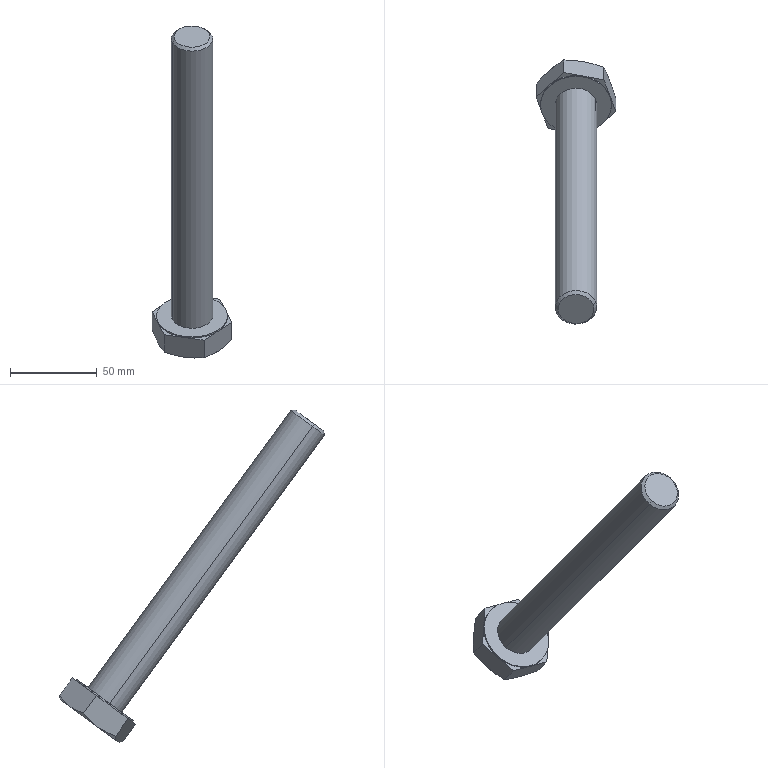Component | SolidWorks | hex structural bolt gradec short_iso-4 | 1 solid | 27 faces | box 46.18 x 152.88 x 191.78 mm | volume 112034 mm3 | plane 15 | cone 8 | cylinder 4 | commonest cylinder face diameters 41 x2 24 x2
STEP:
#1=CARTESIAN_POINT('',(-39.692,28.73,8.663));
#2=VERTEX_POINT('',#1);
#3=CARTESIAN_POINT('',(-38.151,29.116,8.946));
#4=VERTEX_POINT('',#3);
#5=CARTESIAN_POINT('',(-38.921,28.923,8.805));
#6=DIRECTION('',(0.,-0.5907,0.8069));
#7=DIRECTION('',(-0.9549,-0.2396,-0.1754));
#8=AXIS2_PLACEMENT_3D('',#5,#6,#7);
#9=CIRCLE('',#8,0.8071);
#10=EDGE_CURVE('',#2,#4,#9,.T.);
#11=ORIENTED_EDGE('',*,*,#10,.F.);
#12=CARTESIAN_POINT('',(-39.692,28.748,8.638));
#13=VERTEX_POINT('',#12);
#14=CARTESIAN_POINT('',(-39.692,29.079,8.187));
#15=DIRECTION('',(-0.,0.5907,-0.8069));
#16=VECTOR('',#15,39.37);
#17=LINE('',#14,#16);
#18=EDGE_CURVE('',#2,#13,#17,.T.);
#19=ORIENTED_EDGE('',*,*,#18,.T.);
#20=CARTESIAN_POINT('',(-39.099,28.307,8.314));
#21=VERTEX_POINT('',#20);
#22=CARTESIAN_POINT('',(-38.921,28.942,8.779));
#23=DIRECTION('',(-0.,0.5907,-0.8069));
#24=DIRECTION('',(0.9549,0.2396,0.1754));
#25=AXIS2_PLACEMENT_3D('',#22,#23,#24);
#26=CIRCLE('',#25,0.8071);
#27=EDGE_CURVE('',#21,#13,#26,.T.);
#28=ORIENTED_EDGE('',*,*,#27,.F.);
#29=CARTESIAN_POINT('',(-38.328,28.5,8.456));
#30=VERTEX_POINT('',#29);
#31=CARTESIAN_POINT('',(-38.921,28.942,8.779));
#32=DIRECTION('',(-0.,0.5907,-0.8069));
#33=DIRECTION('',(0.9549,0.2396,0.1754));
#34=AXIS2_PLACEMENT_3D('',#31,#32,#33);
#35=CIRCLE('',#34,0.8071);
#36=EDGE_CURVE('',#30,#21,#35,.T.);
#37=ORIENTED_EDGE('',*,*,#36,.F.);
#38=CARTESIAN_POINT('',(-38.151,29.135,8.921));
#39=VERTEX_POINT('',#38);
#40=CARTESIAN_POINT('',(-38.921,28.942,8.779));
#41=DIRECTION('',(-0.,0.5907,-0.8069));
#42=DIRECTION('',(0.9549,0.2396,0.1754));
#43=AXIS2_PLACEMENT_3D('',#40,#41,#42);
#44=CIRCLE('',#43,0.8071);
#45=EDGE_CURVE('',#39,#30,#44,.T.);
#46=ORIENTED_EDGE('',*,*,#45,.F.);
#47=CARTESIAN_POINT('',(-38.151,29.465,8.47));
#48=DIRECTION('',(-0.,0.5907,-0.8069));
#49=VECTOR('',#48,39.37);
#50=LINE('',#47,#49);
#51=EDGE_CURVE('',#4,#39,#50,.T.);
#52=ORIENTED_EDGE('',*,*,#51,.F.);
#53=EDGE_LOOP('',(#11,#19,#28,#37,#46,#52));
#54=FACE_OUTER_BOUND('',#53,.T.);
#55=CARTESIAN_POINT('',(-38.921,29.272,8.328));
#56=DIRECTION('',(-0.,0.5907,-0.8069));
#57=DIRECTION('',(0.9549,0.2396,0.1754));
#58=AXIS2_PLACEMENT_3D('',#55,#56,#57);
#59=CYLINDRICAL_SURFACE('',#58,0.8071);
#60=ADVANCED_FACE('',(#54),#59,.T.);
#61=CARTESIAN_POINT('',(-38.532,24.369,15.229));
#62=VERTEX_POINT('',#61);
#63=CARTESIAN_POINT('',(-39.31,24.174,15.086));
#64=VERTEX_POINT('',#63);
#65=CARTESIAN_POINT('',(-38.921,24.272,15.158));
#66=DIRECTION('',(-0.,0.5907,-0.8069));
#67=DIRECTION('',(0.9549,0.2396,0.1754));
#68=AXIS2_PLACEMENT_3D('',#65,#66,#67);
#69=CIRCLE('',#68,0.4076);
#70=EDGE_CURVE('',#62,#64,#69,.T.);
#71=ORIENTED_EDGE('',*,*,#70,.T.);
#72=CARTESIAN_POINT('',(-39.372,24.197,15.023));
#73=VERTEX_POINT('',#72);
#74=CARTESIAN_POINT('',(-39.31,24.174,15.086));
#75=DIRECTION('',(-0.6752,0.2483,-0.6946));
#76=VECTOR('',#75,39.37);
#77=LINE('',#74,#76);
#78=EDGE_CURVE('',#64,#73,#77,.T.);
#79=ORIENTED_EDGE('',*,*,#78,.T.);
#80=CARTESIAN_POINT('',(-38.47,24.423,15.188));
#81=VERTEX_POINT('',#80);
#82=CARTESIAN_POINT('',(-38.921,24.31,15.105));
#83=DIRECTION('',(-0.,0.5907,-0.8069));
#84=DIRECTION('',(0.9549,0.2396,0.1754));
#85=AXIS2_PLACEMENT_3D('',#82,#83,#84);
#86=CIRCLE('',#85,0.4724);
#87=EDGE_CURVE('',#81,#73,#86,.T.);
#88=ORIENTED_EDGE('',*,*,#87,.F.);
#89=CARTESIAN_POINT('',(-38.532,24.369,15.229));
#90=DIRECTION('',(0.6752,0.5871,-0.4465));
#91=VECTOR('',#90,39.37);
#92=LINE('',#89,#91);
#93=EDGE_CURVE('',#62,#81,#92,.T.);
#94=ORIENTED_EDGE('',*,*,#93,.F.);
#95=EDGE_LOOP('',(#71,#79,#88,#94));
#96=FACE_OUTER_BOUND('',#95,.T.);
#97=CARTESIAN_POINT('',(-38.921,24.272,15.158));
#98=DIRECTION('',(-0.,0.5907,-0.8069));
#99=DIRECTION('',(0.9549,0.2396,0.1754));
#100=AXIS2_PLACEMENT_3D('',#97,#98,#99);
#101=CONICAL_SURFACE('',#100,0.4076,0.7854);
#102=ADVANCED_FACE('',(#96),#101,.T.);
#103=ORIENTED_EDGE('',*,*,#87,.T.);
#104=CARTESIAN_POINT('',(-39.372,28.81,8.722));
#105=VERTEX_POINT('',#104);
#106=CARTESIAN_POINT('',(-39.372,29.159,8.245));
#107=DIRECTION('',(-0.,0.5907,-0.8069));
#108=VECTOR('',#107,39.37);
#109=LINE('',#106,#108);
#110=EDGE_CURVE('',#73,#105,#109,.T.);
#111=ORIENTED_EDGE('',*,*,#110,.T.);
#112=CARTESIAN_POINT('',(-38.47,29.036,8.887));
#113=VERTEX_POINT('',#112);
#114=CARTESIAN_POINT('',(-38.921,28.923,8.805));
#115=DIRECTION('',(-0.,0.5907,-0.8069));
#116=DIRECTION('',(-0.9549,-0.2396,-0.1754));
#117=AXIS2_PLACEMENT_3D('',#114,#115,#116);
#118=CIRCLE('',#117,0.4724);
#119=EDGE_CURVE('',#113,#105,#118,.T.);
#120=ORIENTED_EDGE('',*,*,#119,.F.);
#121=CARTESIAN_POINT('',(-38.47,29.385,8.411));
#122=DIRECTION('',(-0.,0.5907,-0.8069));
#123=VECTOR('',#122,39.37);
#124=LINE('',#121,#123);
#125=EDGE_CURVE('',#81,#113,#124,.T.);
#126=ORIENTED_EDGE('',*,*,#125,.F.);
#127=EDGE_LOOP('',(#103,#111,#120,#126));
#128=FACE_OUTER_BOUND('',#127,.T.);
#129=CARTESIAN_POINT('',(-38.921,29.272,8.328));
#130=DIRECTION('',(-0.,0.5907,-0.8069));
#131=DIRECTION('',(0.9549,0.2396,0.1754));
#132=AXIS2_PLACEMENT_3D('',#129,#130,#131);
#133=CYLINDRICAL_SURFACE('',#132,0.4724);
#134=ADVANCED_FACE('',(#128),#133,.T.);
#135=ORIENTED_EDGE('',*,*,#119,.T.);
#136=CARTESIAN_POINT('',(-38.921,28.923,8.805));
#137=DIRECTION('',(-0.,0.5907,-0.8069));
#138=DIRECTION('',(-0.9549,-0.2396,-0.1754));
#139=AXIS2_PLACEMENT_3D('',#136,#137,#138);
#140=CIRCLE('',#139,0.4724);
#141=EDGE_CURVE('',#105,#113,#140,.T.);
#142=ORIENTED_EDGE('',*,*,#141,.T.);
#143=EDGE_LOOP('',(#135,#142));
#144=FACE_BOUND('',#143,.T.);
#145=CARTESIAN_POINT('',(-38.921,28.923,8.805));
#146=DIRECTION('',(0.,-0.5907,0.8069));
#147=DIRECTION('',(-0.9549,-0.2396,-0.1754));
#148=AXIS2_PLACEMENT_3D('',#145,#146,#147);
#149=CIRCLE('',#148,0.8071);
#150=EDGE_CURVE('',#4,#2,#149,.T.);
#151=ORIENTED_EDGE('',*,*,#150,.T.);
#152=ORIENTED_EDGE('',*,*,#10,.T.);
#153=EDGE_LOOP('',(#151,#152));
#154=FACE_OUTER_BOUND('',#153,.T.);
#155=CARTESIAN_POINT('',(-38.645,28.205,8.279));
#156=DIRECTION('',(0.,-0.5907,0.8069));
#157=DIRECTION('',(-0.9549,-0.2396,-0.1754));
#158=AXIS2_PLACEMENT_3D('',#155,#156,#157);
#159=PLANE('',#158);
#160=ADVANCED_FACE('',(#144,#154),#159,.T.);
#161=ORIENTED_EDGE('',*,*,#110,.F.);
#162=CARTESIAN_POINT('',(-38.921,24.31,15.105));
#163=DIRECTION('',(-0.,0.5907,-0.8069));
#164=DIRECTION('',(0.9549,0.2396,0.1754));
#165=AXIS2_PLACEMENT_3D('',#162,#163,#164);
#166=CIRCLE('',#165,0.4724);
#167=EDGE_CURVE('',#73,#81,#166,.T.);
#168=ORIENTED_EDGE('',*,*,#167,.T.);
#169=ORIENTED_EDGE('',*,*,#125,.T.);
#170=ORIENTED_EDGE('',*,*,#141,.F.);
#171=EDGE_LOOP('',(#161,#168,#169,#170));
#172=FACE_OUTER_BOUND('',#171,.T.);
#173=CARTESIAN_POINT('',(-38.921,29.272,8.328));
#174=DIRECTION('',(-0.,0.5907,-0.8069));
#175=DIRECTION('',(0.9549,0.2396,0.1754));
#176=AXIS2_PLACEMENT_3D('',#173,#174,#175);
#177=CYLINDRICAL_SURFACE('',#176,0.4724);
#178=ADVANCED_FACE('',(#172),#177,.T.);
#179=ORIENTED_EDGE('',*,*,#78,.F.);
#180=CARTESIAN_POINT('',(-38.921,24.272,15.158));
#181=DIRECTION('',(-0.,0.5907,-0.8069));
#182=DIRECTION('',(0.9549,0.2396,0.1754));
#183=AXIS2_PLACEMENT_3D('',#180,#181,#182);
#184=CIRCLE('',#183,0.4076);
#185=EDGE_CURVE('',#64,#62,#184,.T.);
#186=ORIENTED_EDGE('',*,*,#185,.T.);
#187=ORIENTED_EDGE('',*,*,#93,.T.);
#188=ORIENTED_EDGE('',*,*,#167,.F.);
#189=EDGE_LOOP('',(#179,#186,#187,#188));
#190=FACE_OUTER_BOUND('',#189,.T.);
#191=CARTESIAN_POINT('',(-38.921,24.272,15.158));
#192=DIRECTION('',(-0.,0.5907,-0.8069));
#193=DIRECTION('',(0.9549,0.2396,0.1754));
#194=AXIS2_PLACEMENT_3D('',#191,#192,#193);
#195=CONICAL_SURFACE('',#194,0.4076,0.7854);
#196=ADVANCED_FACE('',(#190),#195,.T.);
#197=ORIENTED_EDGE('',*,*,#70,.F.);
#198=ORIENTED_EDGE('',*,*,#185,.F.);
#199=EDGE_LOOP('',(#197,#198));
#200=FACE_OUTER_BOUND('',#199,.T.);
#201=CARTESIAN_POINT('',(-38.921,24.272,15.158));
#202=DIRECTION('',(-0.,0.5907,-0.8069));
#203=DIRECTION('',(0.9549,0.2396,0.1754));
#204=AXIS2_PLACEMENT_3D('',#201,#202,#203);
#205=PLANE('',#204);
#206=ADVANCED_FACE('',(#200),#205,.F.);
#207=CARTESIAN_POINT('',(-39.554,28.389,8.375));
#208=VERTEX_POINT('',#207);
#209=CARTESIAN_POINT('',(-39.554,28.389,8.375));
#210=DIRECTION('',(0.9754,-0.1778,-0.1301));
#211=VECTOR('',#210,39.37);
#212=LINE('',#209,#211);
#213=EDGE_CURVE('',#208,#21,#212,.T.);
#214=ORIENTED_EDGE('',*,*,#213,.T.);
#215=ORIENTED_EDGE('',*,*,#27,.T.);
#216=CARTESIAN_POINT('',(-39.554,28.389,8.375));
#217=DIRECTION('',(0.2969,-0.7705,-0.5641));
#218=VECTOR('',#217,39.37);
#219=LINE('',#216,#218);
#220=EDGE_CURVE('',#13,#208,#219,.T.);
#221=ORIENTED_EDGE('',*,*,#220,.T.);
#222=EDGE_LOOP('',(#214,#215,#221));
#223=FACE_OUTER_BOUND('',#222,.T.);
#224=CARTESIAN_POINT('',(-38.682,28.32,8.324));
#225=DIRECTION('',(0.,-0.5907,0.8069));
#226=DIRECTION('',(-0.9549,-0.2396,-0.1754));
#227=AXIS2_PLACEMENT_3D('',#224,#225,#226);
#228=PLANE('',#227);
#229=ADVANCED_FACE('',(#223),#228,.T.);
#230=CARTESIAN_POINT('',(-38.645,28.224,8.253));
#231=VERTEX_POINT('',#230);
#232=CARTESIAN_POINT('',(-39.554,28.389,8.375));
#233=DIRECTION('',(0.9754,-0.1778,-0.1301));
#234=VECTOR('',#233,39.37);
#235=LINE('',#232,#234);
#236=EDGE_CURVE('',#21,#231,#235,.T.);
#237=ORIENTED_EDGE('',*,*,#236,.T.);
#238=CARTESIAN_POINT('',(-38.645,28.224,8.253));
#239=DIRECTION('',(0.6785,0.5927,0.434));
#240=VECTOR('',#239,39.37);
#241=LINE('',#238,#240);
#242=EDGE_CURVE('',#231,#30,#241,.T.);
#243=ORIENTED_EDGE('',*,*,#242,.T.);
#244=ORIENTED_EDGE('',*,*,#36,.T.);
#245=EDGE_LOOP('',(#237,#243,#244));
#246=FACE_OUTER_BOUND('',#245,.T.);
#247=CARTESIAN_POINT('',(-38.682,28.32,8.324));
#248=DIRECTION('',(0.,-0.5907,0.8069));
#249=DIRECTION('',(-0.9549,-0.2396,-0.1754));
#250=AXIS2_PLACEMENT_3D('',#247,#248,#249);
#251=PLANE('',#250);
#252=ADVANCED_FACE('',(#246),#251,.T.);
#253=CARTESIAN_POINT('',(-38.012,28.776,8.658));
#254=VERTEX_POINT('',#253);
#255=CARTESIAN_POINT('',(-38.645,28.224,8.253));
#256=DIRECTION('',(0.6785,0.5927,0.434));
#257=VECTOR('',#256,39.37);
#258=LINE('',#255,#257);
#259=EDGE_CURVE('',#30,#254,#258,.T.);
#260=ORIENTED_EDGE('',*,*,#259,.T.);
#261=CARTESIAN_POINT('',(-38.012,28.776,8.658));
#262=DIRECTION('',(-0.2969,0.7705,0.5641));
#263=VECTOR('',#262,39.37);
#264=LINE('',#261,#263);
#265=EDGE_CURVE('',#254,#39,#264,.T.);
#266=ORIENTED_EDGE('',*,*,#265,.T.);
#267=ORIENTED_EDGE('',*,*,#45,.T.);
#268=EDGE_LOOP('',(#260,#266,#267));
#269=FACE_OUTER_BOUND('',#268,.T.);
#270=CARTESIAN_POINT('',(-38.682,28.32,8.324));
#271=DIRECTION('',(0.,-0.5907,0.8069));
#272=DIRECTION('',(-0.9549,-0.2396,-0.1754));
#273=AXIS2_PLACEMENT_3D('',#270,#271,#272);
#274=PLANE('',#273);
#275=ADVANCED_FACE('',(#269),#274,.T.);
#276=CARTESIAN_POINT('',(-38.289,29.494,9.184));
#277=VERTEX_POINT('',#276);
#278=CARTESIAN_POINT('',(-38.012,28.776,8.658));
#279=DIRECTION('',(-0.2969,0.7705,0.5641));
#280=VECTOR('',#279,39.37);
#281=LINE('',#278,#280);
#282=EDGE_CURVE('',#39,#277,#281,.T.);
#283=ORIENTED_EDGE('',*,*,#282,.T.);
#284=CARTESIAN_POINT('',(-38.743,29.577,9.244));
#285=VERTEX_POINT('',#284);
#286=CARTESIAN_POINT('',(-39.198,29.66,9.305));
#287=DIRECTION('',(-0.9754,0.1778,0.1301));
#288=VECTOR('',#287,39.37);
#289=LINE('',#286,#288);
#290=EDGE_CURVE('',#277,#285,#289,.T.);
#291=ORIENTED_EDGE('',*,*,#290,.T.);
#292=CARTESIAN_POINT('',(-38.921,28.942,8.779));
#293=DIRECTION('',(-0.,0.5907,-0.8069));
#294=DIRECTION('',(0.9549,0.2396,0.1754));
#295=AXIS2_PLACEMENT_3D('',#292,#293,#294);
#296=CIRCLE('',#295,0.8071);
#297=EDGE_CURVE('',#285,#39,#296,.T.);
#298=ORIENTED_EDGE('',*,*,#297,.T.);
#299=EDGE_LOOP('',(#283,#291,#298));
#300=FACE_OUTER_BOUND('',#299,.T.);
#301=CARTESIAN_POINT('',(-38.682,28.32,8.324));
#302=DIRECTION('',(0.,-0.5907,0.8069));
#303=DIRECTION('',(-0.9549,-0.2396,-0.1754));
#304=AXIS2_PLACEMENT_3D('',#301,#302,#303);
#305=PLANE('',#304);
#306=ADVANCED_FACE('',(#300),#305,.T.);
#307=CARTESIAN_POINT('',(-39.198,29.66,9.305));
#308=VERTEX_POINT('',#307);
#309=CARTESIAN_POINT('',(-39.198,29.66,9.305));
#310=DIRECTION('',(-0.9754,0.1778,0.1301));
#311=VECTOR('',#310,39.37);
#312=LINE('',#309,#311);
#313=EDGE_CURVE('',#285,#308,#312,.T.);
#314=ORIENTED_EDGE('',*,*,#313,.T.);
#315=CARTESIAN_POINT('',(-39.514,29.384,9.103));
#316=VERTEX_POINT('',#315);
#317=CARTESIAN_POINT('',(-39.83,29.107,8.901));
#318=DIRECTION('',(-0.6785,-0.5927,-0.434));
#319=VECTOR('',#318,39.37);
#320=LINE('',#317,#319);
#321=EDGE_CURVE('',#308,#316,#320,.T.);
#322=ORIENTED_EDGE('',*,*,#321,.T.);
#323=CARTESIAN_POINT('',(-38.921,28.942,8.779));
#324=DIRECTION('',(-0.,0.5907,-0.8069));
#325=DIRECTION('',(0.9549,0.2396,0.1754));
#326=AXIS2_PLACEMENT_3D('',#323,#324,#325);
#327=CIRCLE('',#326,0.8071);
#328=EDGE_CURVE('',#316,#285,#327,.T.);
#329=ORIENTED_EDGE('',*,*,#328,.T.);
#330=EDGE_LOOP('',(#314,#322,#329));
#331=FACE_OUTER_BOUND('',#330,.T.);
#332=CARTESIAN_POINT('',(-38.682,28.32,8.324));
#333=DIRECTION('',(0.,-0.5907,0.8069));
#334=DIRECTION('',(-0.9549,-0.2396,-0.1754));
#335=AXIS2_PLACEMENT_3D('',#332,#333,#334);
#336=PLANE('',#335);
#337=ADVANCED_FACE('',(#331),#336,.T.);
#338=CARTESIAN_POINT('',(-39.83,29.107,8.901));
#339=VERTEX_POINT('',#338);
#340=CARTESIAN_POINT('',(-39.83,29.107,8.901));
#341=DIRECTION('',(-0.6785,-0.5927,-0.434));
#342=VECTOR('',#341,39.37);
#343=LINE('',#340,#342);
#344=EDGE_CURVE('',#316,#339,#343,.T.);
#345=ORIENTED_EDGE('',*,*,#344,.T.);
#346=CARTESIAN_POINT('',(-39.554,28.389,8.375));
#347=DIRECTION('',(0.2969,-0.7705,-0.5641));
#348=VECTOR('',#347,39.37);
#349=LINE('',#346,#348);
#350=EDGE_CURVE('',#339,#13,#349,.T.);
#351=ORIENTED_EDGE('',*,*,#350,.T.);
#352=CARTESIAN_POINT('',(-38.921,28.942,8.779));
#353=DIRECTION('',(-0.,0.5907,-0.8069));
#354=DIRECTION('',(0.9549,0.2396,0.1754));
#355=AXIS2_PLACEMENT_3D('',#352,#353,#354);
#356=CIRCLE('',#355,0.8071);
#357=EDGE_CURVE('',#13,#316,#356,.T.);
#358=ORIENTED_EDGE('',*,*,#357,.T.);
#359=EDGE_LOOP('',(#345,#351,#358));
#360=FACE_OUTER_BOUND('',#359,.T.);
#361=CARTESIAN_POINT('',(-38.682,28.32,8.324));
#362=DIRECTION('',(0.,-0.5907,0.8069));
#363=DIRECTION('',(-0.9549,-0.2396,-0.1754));
#364=AXIS2_PLACEMENT_3D('',#361,#362,#363);
#365=PLANE('',#364);
#366=ADVANCED_FACE('',(#360),#365,.T.);
#367=ORIENTED_EDGE('',*,*,#18,.F.);
#368=ORIENTED_EDGE('',*,*,#150,.F.);
#369=ORIENTED_EDGE('',*,*,#51,.T.);
#370=ORIENTED_EDGE('',*,*,#297,.F.);
#371=ORIENTED_EDGE('',*,*,#328,.F.);
#372=ORIENTED_EDGE('',*,*,#357,.F.);
#373=EDGE_LOOP('',(#367,#368,#369,#370,#371,#372));
#374=FACE_OUTER_BOUND('',#373,.T.);
#375=CARTESIAN_POINT('',(-38.921,29.272,8.328));
#376=DIRECTION('',(-0.,0.5907,-0.8069));
#377=DIRECTION('',(0.9549,0.2396,0.1754));
#378=AXIS2_PLACEMENT_3D('',#375,#376,#377);
#379=CYLINDRICAL_SURFACE('',#378,0.8071);
#380=ADVANCED_FACE('',(#374),#379,.T.);
#381=CARTESIAN_POINT('',(-39.692,29.079,8.187));
#382=VERTEX_POINT('',#381);
#383=CARTESIAN_POINT('',(-39.099,28.637,7.863));
#384=VERTEX_POINT('',#383);
#385=CARTESIAN_POINT('',(-38.921,29.272,8.328));
#386=DIRECTION('',(0.,-0.5907,0.8069));
#387=DIRECTION('',(-0.9549,-0.2396,-0.1754));
#388=AXIS2_PLACEMENT_3D('',#385,#386,#387);
#389=CIRCLE('',#388,0.8071);
#390=EDGE_CURVE('',#382,#384,#389,.T.);
#391=ORIENTED_EDGE('',*,*,#390,.F.);
#392=CARTESIAN_POINT('',(-39.514,29.714,8.652));
#393=VERTEX_POINT('',#392);
#394=CARTESIAN_POINT('',(-38.921,29.272,8.328));
#395=DIRECTION('',(0.,-0.5907,0.8069));
#396=DIRECTION('',(-0.9549,-0.2396,-0.1754));
#397=AXIS2_PLACEMENT_3D('',#394,#395,#396);
#398=CIRCLE('',#397,0.8071);
#399=EDGE_CURVE('',#393,#382,#398,.T.);
#400=ORIENTED_EDGE('',*,*,#399,.F.);
#401=CARTESIAN_POINT('',(-38.743,29.907,8.793));
#402=VERTEX_POINT('',#401);
#403=CARTESIAN_POINT('',(-38.921,29.272,8.328));
#404=DIRECTION('',(0.,-0.5907,0.8069));
#405=DIRECTION('',(-0.9549,-0.2396,-0.1754));
#406=AXIS2_PLACEMENT_3D('',#403,#404,#405);
#407=CIRCLE('',#406,0.8071);
#408=EDGE_CURVE('',#402,#393,#407,.T.);
#409=ORIENTED_EDGE('',*,*,#408,.F.);
#410=CARTESIAN_POINT('',(-38.151,29.465,8.47));
#411=VERTEX_POINT('',#410);
#412=CARTESIAN_POINT('',(-38.921,29.272,8.328));
#413=DIRECTION('',(0.,-0.5907,0.8069));
#414=DIRECTION('',(-0.9549,-0.2396,-0.1754));
#415=AXIS2_PLACEMENT_3D('',#412,#413,#414);
#416=CIRCLE('',#415,0.8071);
#417=EDGE_CURVE('',#411,#402,#416,.T.);
#418=ORIENTED_EDGE('',*,*,#417,.F.);
#419=CARTESIAN_POINT('',(-38.328,28.83,8.005));
#420=VERTEX_POINT('',#419);
#421=CARTESIAN_POINT('',(-38.921,29.272,8.328));
#422=DIRECTION('',(-0.,0.5907,-0.8069));
#423=DIRECTION('',(0.9549,0.2396,0.1754));
#424=AXIS2_PLACEMENT_3D('',#421,#422,#423);
#425=CIRCLE('',#424,0.8071);
#426=EDGE_CURVE('',#411,#420,#425,.T.);
#427=ORIENTED_EDGE('',*,*,#426,.T.);
#428=CARTESIAN_POINT('',(-38.921,29.272,8.328));
#429=DIRECTION('',(0.,-0.5907,0.8069));
#430=DIRECTION('',(-0.9549,-0.2396,-0.1754));
#431=AXIS2_PLACEMENT_3D('',#428,#429,#430);
#432=CIRCLE('',#431,0.8071);
#433=EDGE_CURVE('',#384,#420,#432,.T.);
#434=ORIENTED_EDGE('',*,*,#433,.F.);
#435=EDGE_LOOP('',(#391,#400,#409,#418,#427,#434));
#436=FACE_OUTER_BOUND('',#435,.T.);
#437=CARTESIAN_POINT('',(-38.645,28.554,7.802));
#438=DIRECTION('',(0.,-0.5907,0.8069));
#439=DIRECTION('',(-0.9549,-0.2396,-0.1754));
#440=AXIS2_PLACEMENT_3D('',#437,#438,#439);
#441=PLANE('',#440);
#442=ADVANCED_FACE('',(#436),#441,.F.);
#443=CARTESIAN_POINT('',(-38.645,28.511,7.861));
#444=VERTEX_POINT('',#443);
#445=CARTESIAN_POINT('',(-38.328,28.83,8.005));
#446=CARTESIAN_POINT('',(-38.342,28.818,7.996));
#447=CARTESIAN_POINT('',(-38.355,28.806,7.988));
#448=CARTESIAN_POINT('',(-38.382,28.782,7.972));
#449=CARTESIAN_POINT('',(-38.395,28.77,7.964));
#450=CARTESIAN_POINT('',(-38.435,28.732,7.943));
#451=CARTESIAN_POINT('',(-38.462,28.706,7.93));
#452=CARTESIAN_POINT('',(-38.541,28.626,7.895));
#453=CARTESIAN_POINT('',(-38.593,28.569,7.876));
#454=CARTESIAN_POINT('',(-38.645,28.511,7.861));
#455=B_SPLINE_CURVE_WITH_KNOTS('',3,(#445,#446,#447,#448,#449,#450,#451,#452,#453,#454),.UNSPECIFIED.,.F.,.F.,(4,2,2,2,4),(0.01198,0.01347,0.01496,0.01794,0.02391),.UNSPECIFIED.);
#456=EDGE_CURVE('',#420,#444,#455,.T.);
#457=ORIENTED_EDGE('',*,*,#456,.T.);
#458=CARTESIAN_POINT('',(-38.645,28.511,7.861));
#459=CARTESIAN_POINT('',(-38.719,28.538,7.853));
#460=CARTESIAN_POINT('',(-38.794,28.562,7.848));
#461=CARTESIAN_POINT('',(-38.945,28.605,7.848));
#462=CARTESIAN_POINT('',(-39.022,28.623,7.853));
#463=CARTESIAN_POINT('',(-39.099,28.637,7.863));
#464=B_SPLINE_CURVE_WITH_KNOTS('',3,(#458,#459,#460,#461,#462,#463),.UNSPECIFIED.,.F.,.F.,(4,2,4),(0.00000024,0.005988,0.01198),.UNSPECIFIED.);
#465=EDGE_CURVE('',#444,#384,#464,.T.);
#466=ORIENTED_EDGE('',*,*,#465,.T.);
#467=ORIENTED_EDGE('',*,*,#433,.T.);
#468=EDGE_LOOP('',(#457,#466,#467));
#469=FACE_OUTER_BOUND('',#468,.T.);
#470=CARTESIAN_POINT('',(-38.921,29.272,8.328));
#471=DIRECTION('',(0.,-0.5907,0.8069));
#472=DIRECTION('',(-0.9549,-0.2396,-0.1754));
#473=AXIS2_PLACEMENT_3D('',#470,#471,#472);
#474=CONICAL_SURFACE('',#473,0.8071,1.047);
#475=ADVANCED_FACE('',(#469),#474,.T.);
#476=CARTESIAN_POINT('',(-38.012,29.064,8.265));
#477=VERTEX_POINT('',#476);
#478=CARTESIAN_POINT('',(-38.151,29.465,8.47));
#479=CARTESIAN_POINT('',(-38.139,29.435,8.447));
#480=CARTESIAN_POINT('',(-38.127,29.403,8.426));
#481=CARTESIAN_POINT('',(-38.104,29.338,8.387));
#482=CARTESIAN_POINT('',(-38.092,29.305,8.369));
#483=CARTESIAN_POINT('',(-38.057,29.204,8.318));
#484=CARTESIAN_POINT('',(-38.035,29.135,8.29));
#485=CARTESIAN_POINT('',(-38.012,29.064,8.265));
#486=B_SPLINE_CURVE_WITH_KNOTS('',3,(#478,#479,#480,#481,#482,#483,#484,#485),.UNSPECIFIED.,.F.,.F.,(4,2,2,4),(0.03354,0.03654,0.03953,0.04553),.UNSPECIFIED.);
#487=EDGE_CURVE('',#411,#477,#486,.T.);
#488=ORIENTED_EDGE('',*,*,#487,.T.);
#489=CARTESIAN_POINT('',(-38.012,29.064,8.265));
#490=CARTESIAN_POINT('',(-38.064,29.032,8.214));
#491=CARTESIAN_POINT('',(-38.116,28.997,8.166));
#492=CARTESIAN_POINT('',(-38.221,28.92,8.079));
#493=CARTESIAN_POINT('',(-38.275,28.877,8.039));
#494=CARTESIAN_POINT('',(-38.328,28.83,8.005));
#495=B_SPLINE_CURVE_WITH_KNOTS('',3,(#489,#490,#491,#492,#493,#494),.UNSPECIFIED.,.F.,.F.,(4,2,4),(0.00000024,0.005988,0.01198),.UNSPECIFIED.);
#496=EDGE_CURVE('',#477,#420,#495,.T.);
#497=ORIENTED_EDGE('',*,*,#496,.T.);
#498=ORIENTED_EDGE('',*,*,#426,.F.);
#499=EDGE_LOOP('',(#488,#497,#498));
#500=FACE_OUTER_BOUND('',#499,.T.);
#501=CARTESIAN_POINT('',(-38.921,29.272,8.328));
#502=DIRECTION('',(0.,-0.5907,0.8069));
#503=DIRECTION('',(-0.9549,-0.2396,-0.1754));
#504=AXIS2_PLACEMENT_3D('',#501,#502,#503);
#505=CONICAL_SURFACE('',#504,0.8071,1.047);
#506=ADVANCED_FACE('',(#500),#505,.T.);
#507=CARTESIAN_POINT('',(-38.289,29.782,8.791));
#508=VERTEX_POINT('',#507);
#509=CARTESIAN_POINT('',(-38.289,29.782,8.791));
#510=CARTESIAN_POINT('',(-38.278,29.759,8.761));
#511=CARTESIAN_POINT('',(-38.266,29.735,8.731));
#512=CARTESIAN_POINT('',(-38.243,29.686,8.673));
#513=CARTESIAN_POINT('',(-38.232,29.661,8.645));
#514=CARTESIAN_POINT('',(-38.197,29.582,8.564));
#515=CARTESIAN_POINT('',(-38.174,29.526,8.514));
#516=CARTESIAN_POINT('',(-38.151,29.465,8.47));
#517=B_SPLINE_CURVE_WITH_KNOTS('',3,(#509,#510,#511,#512,#513,#514,#515,#516),.UNSPECIFIED.,.F.,.F.,(4,2,2,4),(0.02156,0.02456,0.02755,0.03354),.UNSPECIFIED.);
#518=EDGE_CURVE('',#508,#411,#517,.T.);
#519=ORIENTED_EDGE('',*,*,#518,.T.);
#520=ORIENTED_EDGE('',*,*,#417,.T.);
#521=CARTESIAN_POINT('',(-38.743,29.907,8.793));
#522=CARTESIAN_POINT('',(-38.724,29.904,8.791));
#523=CARTESIAN_POINT('',(-38.705,29.9,8.788));
#524=CARTESIAN_POINT('',(-38.666,29.892,8.785));
#525=CARTESIAN_POINT('',(-38.647,29.888,8.783));
#526=CARTESIAN_POINT('',(-38.589,29.874,8.779));
#527=CARTESIAN_POINT('',(-38.551,29.864,8.778));
#528=CARTESIAN_POINT('',(-38.438,29.833,8.778));
#529=CARTESIAN_POINT('',(-38.363,29.808,8.783));
#530=CARTESIAN_POINT('',(-38.289,29.782,8.791));
#531=B_SPLINE_CURVE_WITH_KNOTS('',3,(#521,#522,#523,#524,#525,#526,#527,#528,#529,#530),.UNSPECIFIED.,.F.,.F.,(4,2,2,2,4),(0.01198,0.01347,0.01496,0.01794,0.02391),.UNSPECIFIED.);
#532=EDGE_CURVE('',#402,#508,#531,.T.);
#533=ORIENTED_EDGE('',*,*,#532,.T.);
#534=EDGE_LOOP('',(#519,#520,#533));
#535=FACE_OUTER_BOUND('',#534,.T.);
#536=CARTESIAN_POINT('',(-38.921,29.272,8.328));
#537=DIRECTION('',(0.,-0.5907,0.8069));
#538=DIRECTION('',(-0.9549,-0.2396,-0.1754));
#539=AXIS2_PLACEMENT_3D('',#536,#537,#538);
#540=CONICAL_SURFACE('',#539,0.8071,1.047);
#541=ADVANCED_FACE('',(#535),#540,.T.);
#542=CARTESIAN_POINT('',(-39.198,29.947,8.912));
#543=VERTEX_POINT('',#542);
#544=CARTESIAN_POINT('',(-39.198,29.947,8.912));
#545=CARTESIAN_POINT('',(-39.124,29.947,8.884));
#546=CARTESIAN_POINT('',(-39.049,29.944,8.86));
#547=CARTESIAN_POINT('',(-38.897,29.931,8.819));
#548=CARTESIAN_POINT('',(-38.821,29.921,8.804));
#549=CARTESIAN_POINT('',(-38.743,29.907,8.793));
#550=B_SPLINE_CURVE_WITH_KNOTS('',3,(#544,#545,#546,#547,#548,#549),.UNSPECIFIED.,.F.,.F.,(4,2,4),(0.00000024,0.005988,0.01198),.UNSPECIFIED.);
#551=EDGE_CURVE('',#543,#402,#550,.T.);
#552=ORIENTED_EDGE('',*,*,#551,.T.);
#553=ORIENTED_EDGE('',*,*,#408,.T.);
#554=CARTESIAN_POINT('',(-39.514,29.714,8.652));
#555=CARTESIAN_POINT('',(-39.501,29.726,8.66));
#556=CARTESIAN_POINT('',(-39.487,29.737,8.669));
#557=CARTESIAN_POINT('',(-39.46,29.76,8.688));
#558=CARTESIAN_POINT('',(-39.447,29.77,8.697));
#559=CARTESIAN_POINT('',(-39.407,29.802,8.727));
#560=CARTESIAN_POINT('',(-39.381,29.823,8.748));
#561=CARTESIAN_POINT('',(-39.302,29.881,8.813));
#562=CARTESIAN_POINT('',(-39.25,29.915,8.861));
#563=CARTESIAN_POINT('',(-39.198,29.947,8.912));
#564=B_SPLINE_CURVE_WITH_KNOTS('',3,(#554,#555,#556,#557,#558,#559,#560,#561,#562,#563),.UNSPECIFIED.,.F.,.F.,(4,2,2,2,4),(0.01198,0.01347,0.01496,0.01794,0.02391),.UNSPECIFIED.);
#565=EDGE_CURVE('',#393,#543,#564,.T.);
#566=ORIENTED_EDGE('',*,*,#565,.T.);
#567=EDGE_LOOP('',(#552,#553,#566));
#568=FACE_OUTER_BOUND('',#567,.T.);
#569=CARTESIAN_POINT('',(-38.921,29.272,8.328));
#570=DIRECTION('',(0.,-0.5907,0.8069));
#571=DIRECTION('',(-0.9549,-0.2396,-0.1754));
#572=AXIS2_PLACEMENT_3D('',#569,#570,#571);
#573=CONICAL_SURFACE('',#572,0.8071,1.047);
#574=ADVANCED_FACE('',(#568),#573,.T.);
#575=CARTESIAN_POINT('',(-39.554,28.677,7.982));
#576=VERTEX_POINT('',#575);
#577=CARTESIAN_POINT('',(-39.099,28.637,7.863));
#578=CARTESIAN_POINT('',(-39.118,28.64,7.866));
#579=CARTESIAN_POINT('',(-39.138,28.644,7.869));
#580=CARTESIAN_POINT('',(-39.176,28.65,7.875));
#581=CARTESIAN_POINT('',(-39.196,28.652,7.879));
#582=CARTESIAN_POINT('',(-39.253,28.66,7.89));
#583=CARTESIAN_POINT('',(-39.291,28.664,7.899));
#584=CARTESIAN_POINT('',(-39.405,28.674,7.93));
#585=CARTESIAN_POINT('',(-39.479,28.676,7.954));
#586=CARTESIAN_POINT('',(-39.554,28.677,7.982));
#587=B_SPLINE_CURVE_WITH_KNOTS('',3,(#577,#578,#579,#580,#581,#582,#583,#584,#585,#586),.UNSPECIFIED.,.F.,.F.,(4,2,2,2,4),(0.01198,0.01347,0.01496,0.01794,0.02391),.UNSPECIFIED.);
#588=EDGE_CURVE('',#384,#576,#587,.T.);
#589=ORIENTED_EDGE('',*,*,#588,.T.);
#590=CARTESIAN_POINT('',(-39.554,28.677,7.982));
#591=CARTESIAN_POINT('',(-39.576,28.748,8.007));
#592=CARTESIAN_POINT('',(-39.599,28.817,8.035));
#593=CARTESIAN_POINT('',(-39.633,28.919,8.086));
#594=CARTESIAN_POINT('',(-39.645,28.952,8.104));
#595=CARTESIAN_POINT('',(-39.668,29.017,8.143));
#596=CARTESIAN_POINT('',(-39.68,29.048,8.164));
#597=CARTESIAN_POINT('',(-39.692,29.079,8.187));
#598=B_SPLINE_CURVE_WITH_KNOTS('',3,(#590,#591,#592,#593,#594,#595,#596,#597),.UNSPECIFIED.,.F.,.F.,(4,2,2,4),(0.0533,0.05929,0.06229,0.06529),.UNSPECIFIED.);
#599=EDGE_CURVE('',#576,#382,#598,.T.);
#600=ORIENTED_EDGE('',*,*,#599,.T.);
#601=ORIENTED_EDGE('',*,*,#390,.T.);
#602=EDGE_LOOP('',(#589,#600,#601));
#603=FACE_OUTER_BOUND('',#602,.T.);
#604=CARTESIAN_POINT('',(-38.921,29.272,8.328));
#605=DIRECTION('',(0.,-0.5907,0.8069));
#606=DIRECTION('',(-0.9549,-0.2396,-0.1754));
#607=AXIS2_PLACEMENT_3D('',#604,#605,#606);
#608=CONICAL_SURFACE('',#607,0.8071,1.047);
#609=ADVANCED_FACE('',(#603),#608,.T.);
#610=CARTESIAN_POINT('',(-39.83,29.395,8.508));
#611=VERTEX_POINT('',#610);
#612=CARTESIAN_POINT('',(-39.83,29.395,8.508));
#613=CARTESIAN_POINT('',(-39.779,29.453,8.523));
#614=CARTESIAN_POINT('',(-39.726,29.509,8.542));
#615=CARTESIAN_POINT('',(-39.621,29.616,8.589));
#616=CARTESIAN_POINT('',(-39.568,29.667,8.617));
#617=CARTESIAN_POINT('',(-39.514,29.714,8.652));
#618=B_SPLINE_CURVE_WITH_KNOTS('',3,(#612,#613,#614,#615,#616,#617),.UNSPECIFIED.,.F.,.F.,(4,2,4),(0.00000024,0.005988,0.01198),.UNSPECIFIED.);
#619=EDGE_CURVE('',#611,#393,#618,.T.);
#620=ORIENTED_EDGE('',*,*,#619,.T.);
#621=ORIENTED_EDGE('',*,*,#399,.T.);
#622=CARTESIAN_POINT('',(-39.692,29.079,8.187));
#623=CARTESIAN_POINT('',(-39.715,29.139,8.231));
#624=CARTESIAN_POINT('',(-39.739,29.196,8.281));
#625=CARTESIAN_POINT('',(-39.773,29.274,8.362));
#626=CARTESIAN_POINT('',(-39.785,29.3,8.39));
#627=CARTESIAN_POINT('',(-39.808,29.349,8.448));
#628=CARTESIAN_POINT('',(-39.819,29.372,8.477));
#629=CARTESIAN_POINT('',(-39.83,29.395,8.508));
#630=B_SPLINE_CURVE_WITH_KNOTS('',3,(#622,#623,#624,#625,#626,#627,#628,#629),.UNSPECIFIED.,.F.,.F.,(4,2,2,4),(0.06529,0.07128,0.07428,0.07728),.UNSPECIFIED.);
#631=EDGE_CURVE('',#382,#611,#630,.T.);
#632=ORIENTED_EDGE('',*,*,#631,.T.);
#633=EDGE_LOOP('',(#620,#621,#632));
#634=FACE_OUTER_BOUND('',#633,.T.);
#635=CARTESIAN_POINT('',(-38.921,29.272,8.328));
#636=DIRECTION('',(0.,-0.5907,0.8069));
#637=DIRECTION('',(-0.9549,-0.2396,-0.1754));
#638=AXIS2_PLACEMENT_3D('',#635,#636,#637);
#639=CONICAL_SURFACE('',#638,0.8071,1.047);
#640=ADVANCED_FACE('',(#634),#639,.T.);
#641=ORIENTED_EDGE('',*,*,#350,.F.);
#642=CARTESIAN_POINT('',(-39.83,29.089,8.926));
#643=DIRECTION('',(-0.,0.5907,-0.8069));
#644=VECTOR('',#643,39.37);
#645=LINE('',#642,#644);
#646=EDGE_CURVE('',#339,#611,#645,.T.);
#647=ORIENTED_EDGE('',*,*,#646,.T.);
#648=ORIENTED_EDGE('',*,*,#631,.F.);
#649=ORIENTED_EDGE('',*,*,#599,.F.);
#650=CARTESIAN_POINT('',(-39.554,28.371,8.4));
#651=DIRECTION('',(-0.,0.5907,-0.8069));
#652=VECTOR('',#651,39.37);
#653=LINE('',#650,#652);
#654=EDGE_CURVE('',#208,#576,#653,.T.);
#655=ORIENTED_EDGE('',*,*,#654,.F.);
#656=ORIENTED_EDGE('',*,*,#220,.F.);
#657=EDGE_LOOP('',(#641,#647,#648,#649,#655,#656));
#658=FACE_OUTER_BOUND('',#657,.T.);
#659=CARTESIAN_POINT('',(-39.554,28.371,8.4));
#660=DIRECTION('',(0.9549,0.2396,0.1754));
#661=DIRECTION('',(-0.2969,0.7705,0.5641));
#662=AXIS2_PLACEMENT_3D('',#659,#660,#661);
#663=PLANE('',#662);
#664=ADVANCED_FACE('',(#658),#663,.F.);
#665=ORIENTED_EDGE('',*,*,#321,.F.);
#666=CARTESIAN_POINT('',(-39.198,29.641,9.33));
#667=DIRECTION('',(-0.,0.5907,-0.8069));
#668=VECTOR('',#667,39.37);
#669=LINE('',#666,#668);
#670=EDGE_CURVE('',#308,#543,#669,.T.);
#671=ORIENTED_EDGE('',*,*,#670,.T.);
#672=ORIENTED_EDGE('',*,*,#565,.F.);
#673=ORIENTED_EDGE('',*,*,#619,.F.);
#674=ORIENTED_EDGE('',*,*,#646,.F.);
#675=ORIENTED_EDGE('',*,*,#344,.F.);
#676=EDGE_LOOP('',(#665,#671,#672,#673,#674,#675));
#677=FACE_OUTER_BOUND('',#676,.T.);
#678=CARTESIAN_POINT('',(-39.83,29.089,8.926));
#679=DIRECTION('',(0.7346,-0.5475,-0.4008));
#680=DIRECTION('',(0.6785,0.5927,0.434));
#681=AXIS2_PLACEMENT_3D('',#678,#679,#680);
#682=PLANE('',#681);
#683=ADVANCED_FACE('',(#677),#682,.F.);
#684=ORIENTED_EDGE('',*,*,#290,.F.);
#685=CARTESIAN_POINT('',(-38.289,29.475,9.209));
#686=DIRECTION('',(-0.,0.5907,-0.8069));
#687=VECTOR('',#686,39.37);
#688=LINE('',#685,#687);
#689=EDGE_CURVE('',#277,#508,#688,.T.);
#690=ORIENTED_EDGE('',*,*,#689,.T.);
#691=ORIENTED_EDGE('',*,*,#532,.F.);
#692=ORIENTED_EDGE('',*,*,#551,.F.);
#693=ORIENTED_EDGE('',*,*,#670,.F.);
#694=ORIENTED_EDGE('',*,*,#313,.F.);
#695=EDGE_LOOP('',(#684,#690,#691,#692,#693,#694));
#696=FACE_OUTER_BOUND('',#695,.T.);
#697=CARTESIAN_POINT('',(-39.198,29.641,9.33));
#698=DIRECTION('',(-0.2203,-0.787,-0.5762));
#699=DIRECTION('',(0.9754,-0.1778,-0.1301));
#700=AXIS2_PLACEMENT_3D('',#697,#698,#699);
#701=PLANE('',#700);
#702=ADVANCED_FACE('',(#696),#701,.F.);
#703=ORIENTED_EDGE('',*,*,#265,.F.);
#704=CARTESIAN_POINT('',(-38.012,28.757,8.683));
#705=DIRECTION('',(-0.,0.5907,-0.8069));
#706=VECTOR('',#705,39.37);
#707=LINE('',#704,#706);
#708=EDGE_CURVE('',#254,#477,#707,.T.);
#709=ORIENTED_EDGE('',*,*,#708,.T.);
#710=ORIENTED_EDGE('',*,*,#487,.F.);
#711=ORIENTED_EDGE('',*,*,#518,.F.);
#712=ORIENTED_EDGE('',*,*,#689,.F.);
#713=ORIENTED_EDGE('',*,*,#282,.F.);
#714=EDGE_LOOP('',(#703,#709,#710,#711,#712,#713));
#715=FACE_OUTER_BOUND('',#714,.T.);
#716=CARTESIAN_POINT('',(-38.012,28.757,8.683));
#717=DIRECTION('',(-0.9549,-0.2396,-0.1754));
#718=DIRECTION('',(0.2969,-0.7705,-0.5641));
#719=AXIS2_PLACEMENT_3D('',#716,#717,#718);
#720=PLANE('',#719);
#721=ADVANCED_FACE('',(#715),#720,.F.);
#722=ORIENTED_EDGE('',*,*,#242,.F.);
#723=CARTESIAN_POINT('',(-38.645,28.205,8.279));
#724=DIRECTION('',(-0.,0.5907,-0.8069));
#725=VECTOR('',#724,39.37);
#726=LINE('',#723,#725);
#727=EDGE_CURVE('',#231,#444,#726,.T.);
#728=ORIENTED_EDGE('',*,*,#727,.T.);
#729=ORIENTED_EDGE('',*,*,#456,.F.);
#730=ORIENTED_EDGE('',*,*,#496,.F.);
#731=ORIENTED_EDGE('',*,*,#708,.F.);
#732=ORIENTED_EDGE('',*,*,#259,.F.);
#733=EDGE_LOOP('',(#722,#728,#729,#730,#731,#732));
#734=FACE_OUTER_BOUND('',#733,.T.);
#735=CARTESIAN_POINT('',(-38.645,28.205,8.279));
#736=DIRECTION('',(-0.7346,0.5475,0.4008));
#737=DIRECTION('',(-0.6785,-0.5927,-0.434));
#738=AXIS2_PLACEMENT_3D('',#735,#736,#737);
#739=PLANE('',#738);
#740=ADVANCED_FACE('',(#734),#739,.F.);
#741=ORIENTED_EDGE('',*,*,#213,.F.);
#742=ORIENTED_EDGE('',*,*,#654,.T.);
#743=ORIENTED_EDGE('',*,*,#588,.F.);
#744=ORIENTED_EDGE('',*,*,#465,.F.);
#745=ORIENTED_EDGE('',*,*,#727,.F.);
#746=ORIENTED_EDGE('',*,*,#236,.F.);
#747=EDGE_LOOP('',(#741,#742,#743,#744,#745,#746));
#748=FACE_OUTER_BOUND('',#747,.T.);
#749=CARTESIAN_POINT('',(-39.554,28.371,8.4));
#750=DIRECTION('',(0.2203,0.787,0.5762));
#751=DIRECTION('',(-0.9754,0.1778,0.1301));
#752=AXIS2_PLACEMENT_3D('',#749,#750,#751);
#753=PLANE('',#752);
#754=ADVANCED_FACE('',(#748),#753,.F.);
#755=CLOSED_SHELL('',(#60,#102,#134,#160,#178,#196,#206,#229,#252,#275,#306,#337,#366,#380,#442,#475,#506,#541,#574,#609,#640,#664,#683,#702,#721,#740,#754));
#756=MANIFOLD_SOLID_BREP('',#755);
#757=CARTESIAN_POINT('',(0.,0.,0.));
#758=DIRECTION('',(0.,0.,1.));
#759=DIRECTION('',(1.,0.,0.));
#760=AXIS2_PLACEMENT_3D('',#757,#758,#759);
#761=(LENGTH_UNIT()NAMED_UNIT(*)SI_UNIT($,.METRE.));
#762=LENGTH_MEASURE_WITH_UNIT(LENGTH_MEASURE(0.0254),#761);
#763=DIMENSIONAL_EXPONENTS(1.,0.,0.,0.,0.,0.,0.);
#764=(CONVERSION_BASED_UNIT('',#762)LENGTH_UNIT()NAMED_UNIT(#763));
#765=UNCERTAINTY_MEASURE_WITH_UNIT(LENGTH_MEASURE(0.00001),#764,'','');
#766=(NAMED_UNIT(*)PLANE_ANGLE_UNIT()SI_UNIT($,.RADIAN.));
#767=(NAMED_UNIT(*)SI_UNIT($,.STERADIAN.)SOLID_ANGLE_UNIT());
#768=(GEOMETRIC_REPRESENTATION_CONTEXT(3)GLOBAL_UNCERTAINTY_ASSIGNED_CONTEXT((#765))GLOBAL_UNIT_ASSIGNED_CONTEXT((#764,#766,#767))REPRESENTATION_CONTEXT('',''));
#769=ADVANCED_BREP_SHAPE_REPRESENTATION('',(#756,#760),#768);
#770=COLOUR_RGB('',0.7922,0.8196,0.9333);
#771=FILL_AREA_STYLE_COLOUR('',#770);
#772=FILL_AREA_STYLE('',(#771));
#773=SURFACE_STYLE_FILL_AREA(#772);
#774=SURFACE_SIDE_STYLE('',(#773));
#775=SURFACE_STYLE_USAGE(.BOTH.,#774);
#776=PRESENTATION_STYLE_ASSIGNMENT((#775));
#777=STYLED_ITEM('',(#776),#756);
#778=(LENGTH_UNIT()NAMED_UNIT(*)SI_UNIT($,.METRE.));
#779=LENGTH_MEASURE_WITH_UNIT(LENGTH_MEASURE(0.0254),#778);
#780=DIMENSIONAL_EXPONENTS(1.,0.,0.,0.,0.,0.,0.);
#781=(CONVERSION_BASED_UNIT('',#779)LENGTH_UNIT()NAMED_UNIT(#780));
#782=UNCERTAINTY_MEASURE_WITH_UNIT(LENGTH_MEASURE(0.00001),#781,'','');
#783=(NAMED_UNIT(*)PLANE_ANGLE_UNIT()SI_UNIT($,.RADIAN.));
#784=(NAMED_UNIT(*)SI_UNIT($,.STERADIAN.)SOLID_ANGLE_UNIT());
#785=(GEOMETRIC_REPRESENTATION_CONTEXT(3)GLOBAL_UNCERTAINTY_ASSIGNED_CONTEXT((#782))GLOBAL_UNIT_ASSIGNED_CONTEXT((#781,#783,#784))REPRESENTATION_CONTEXT('',''));
#786=MECHANICAL_DESIGN_GEOMETRIC_PRESENTATION_REPRESENTATION('',(#777),#785);
#787=PRESENTATION_LAYER_ASSIGNMENT('','',(#777));